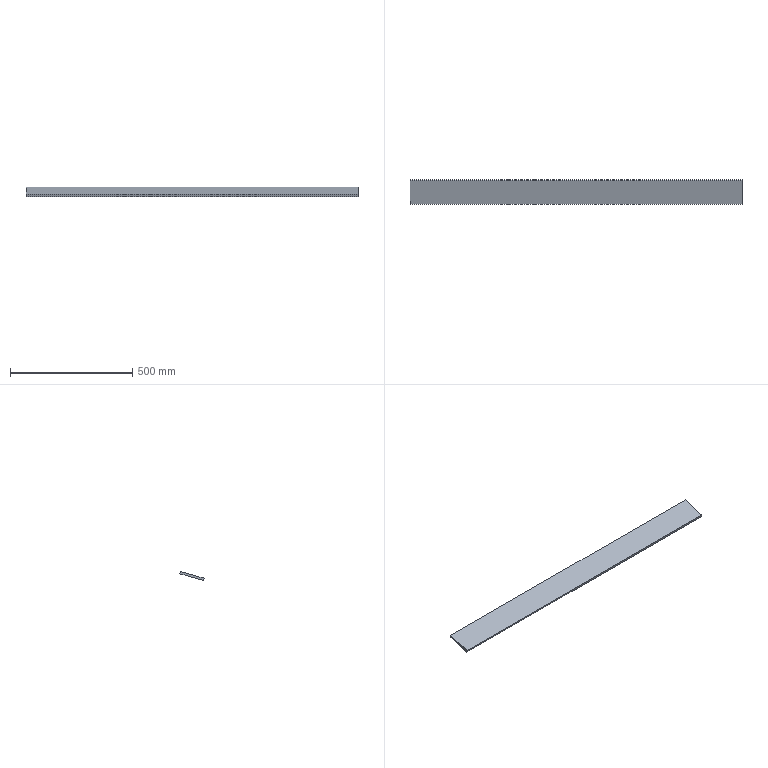Component | SolidWorks | Vezni lim 1-2 | 1 solid | 6 faces | box 1360 x 98.8 x 37.58 mm | volume 1360000 mm3 | plane 6
build123d program:
from build123d import *

# Parameters (mm, degrees)
SKETCH1_W           = 10
SKETCH1_H           = 100
BOSS_EXTRUDE1_DEPTH = 1360


with BuildPart() as part:
    # Sketch1 → Boss-Extrude1 (new body)
    with BuildSketch(Plane.XY):
        with Locations((-108.521, 110)):
            Rectangle(SKETCH1_W, SKETCH1_H)
    extrude(amount=-BOSS_EXTRUDE1_DEPTH)


solid = part.part

# Placed as in the assembly
solid = solid.moved(Location((-1313.6, 1002.358, 806.215), (16.245, -90, 0)))
STEP:
#1=CARTESIAN_POINT('',(1.827,42.981,28.111));
#2=VERTEX_POINT('',#1);
#3=CARTESIAN_POINT('',(1.827,46.761,29.212));
#4=VERTEX_POINT('',#3);
#5=CARTESIAN_POINT('',(1.827,46.761,29.212));
#6=DIRECTION('',(-0.,0.9601,0.2797));
#7=VECTOR('',#6,39.37);
#8=LINE('',#5,#7);
#9=EDGE_CURVE('',#2,#4,#8,.T.);
#10=ORIENTED_EDGE('',*,*,#9,.F.);
#11=CARTESIAN_POINT('',(-51.717,42.981,28.111));
#12=VERTEX_POINT('',#11);
#13=CARTESIAN_POINT('',(-51.717,42.981,28.111));
#14=DIRECTION('',(1.,0.,0.));
#15=VECTOR('',#14,39.37);
#16=LINE('',#13,#15);
#17=EDGE_CURVE('',#12,#2,#16,.T.);
#18=ORIENTED_EDGE('',*,*,#17,.F.);
#19=CARTESIAN_POINT('',(-51.717,46.761,29.212));
#20=VERTEX_POINT('',#19);
#21=CARTESIAN_POINT('',(-51.717,46.761,29.212));
#22=DIRECTION('',(-0.,0.9601,0.2797));
#23=VECTOR('',#22,39.37);
#24=LINE('',#21,#23);
#25=EDGE_CURVE('',#12,#20,#24,.T.);
#26=ORIENTED_EDGE('',*,*,#25,.T.);
#27=CARTESIAN_POINT('',(-51.717,46.761,29.212));
#28=DIRECTION('',(1.,0.,0.));
#29=VECTOR('',#28,39.37);
#30=LINE('',#27,#29);
#31=EDGE_CURVE('',#20,#4,#30,.T.);
#32=ORIENTED_EDGE('',*,*,#31,.T.);
#33=EDGE_LOOP('',(#10,#18,#26,#32));
#34=FACE_OUTER_BOUND('',#33,.T.);
#35=CARTESIAN_POINT('',(-51.717,46.761,29.212));
#36=DIRECTION('',(0.,0.2797,-0.9601));
#37=DIRECTION('',(-1.,-0.,-0.));
#38=AXIS2_PLACEMENT_3D('',#35,#36,#37);
#39=PLANE('',#38);
#40=ADVANCED_FACE('',(#34),#39,.T.);
#41=CARTESIAN_POINT('',(1.827,42.871,28.489));
#42=VERTEX_POINT('',#41);
#43=CARTESIAN_POINT('',(1.827,42.981,28.111));
#44=DIRECTION('',(0.,0.2797,-0.9601));
#45=VECTOR('',#44,39.37);
#46=LINE('',#43,#45);
#47=EDGE_CURVE('',#42,#2,#46,.T.);
#48=ORIENTED_EDGE('',*,*,#47,.F.);
#49=CARTESIAN_POINT('',(-51.717,42.871,28.489));
#50=VERTEX_POINT('',#49);
#51=CARTESIAN_POINT('',(-51.717,42.871,28.489));
#52=DIRECTION('',(1.,0.,0.));
#53=VECTOR('',#52,39.37);
#54=LINE('',#51,#53);
#55=EDGE_CURVE('',#50,#42,#54,.T.);
#56=ORIENTED_EDGE('',*,*,#55,.F.);
#57=CARTESIAN_POINT('',(-51.717,42.981,28.111));
#58=DIRECTION('',(0.,0.2797,-0.9601));
#59=VECTOR('',#58,39.37);
#60=LINE('',#57,#59);
#61=EDGE_CURVE('',#50,#12,#60,.T.);
#62=ORIENTED_EDGE('',*,*,#61,.T.);
#63=ORIENTED_EDGE('',*,*,#17,.T.);
#64=EDGE_LOOP('',(#48,#56,#62,#63));
#65=FACE_OUTER_BOUND('',#64,.T.);
#66=CARTESIAN_POINT('',(-51.717,42.981,28.111));
#67=DIRECTION('',(0.,-0.9601,-0.2797));
#68=DIRECTION('',(-1.,-0.,-0.));
#69=AXIS2_PLACEMENT_3D('',#66,#67,#68);
#70=PLANE('',#69);
#71=ADVANCED_FACE('',(#65),#70,.T.);
#72=CARTESIAN_POINT('',(1.827,46.651,29.59));
#73=VERTEX_POINT('',#72);
#74=CARTESIAN_POINT('',(1.827,46.651,29.59));
#75=DIRECTION('',(0.,-0.9601,-0.2797));
#76=VECTOR('',#75,39.37);
#77=LINE('',#74,#76);
#78=EDGE_CURVE('',#73,#42,#77,.T.);
#79=ORIENTED_EDGE('',*,*,#78,.F.);
#80=CARTESIAN_POINT('',(-51.717,46.651,29.59));
#81=VERTEX_POINT('',#80);
#82=CARTESIAN_POINT('',(-51.717,46.651,29.59));
#83=DIRECTION('',(1.,0.,0.));
#84=VECTOR('',#83,39.37);
#85=LINE('',#82,#84);
#86=EDGE_CURVE('',#81,#73,#85,.T.);
#87=ORIENTED_EDGE('',*,*,#86,.F.);
#88=CARTESIAN_POINT('',(-51.717,46.651,29.59));
#89=DIRECTION('',(0.,-0.9601,-0.2797));
#90=VECTOR('',#89,39.37);
#91=LINE('',#88,#90);
#92=EDGE_CURVE('',#81,#50,#91,.T.);
#93=ORIENTED_EDGE('',*,*,#92,.T.);
#94=ORIENTED_EDGE('',*,*,#55,.T.);
#95=EDGE_LOOP('',(#79,#87,#93,#94));
#96=FACE_OUTER_BOUND('',#95,.T.);
#97=CARTESIAN_POINT('',(-51.717,46.651,29.59));
#98=DIRECTION('',(-0.,-0.2797,0.9601));
#99=DIRECTION('',(0.,-0.9601,-0.2797));
#100=AXIS2_PLACEMENT_3D('',#97,#98,#99);
#101=PLANE('',#100);
#102=ADVANCED_FACE('',(#96),#101,.T.);
#103=CARTESIAN_POINT('',(1.827,46.761,29.212));
#104=DIRECTION('',(-0.,-0.2797,0.9601));
#105=VECTOR('',#104,39.37);
#106=LINE('',#103,#105);
#107=EDGE_CURVE('',#4,#73,#106,.T.);
#108=ORIENTED_EDGE('',*,*,#107,.F.);
#109=ORIENTED_EDGE('',*,*,#31,.F.);
#110=CARTESIAN_POINT('',(-51.717,46.761,29.212));
#111=DIRECTION('',(-0.,-0.2797,0.9601));
#112=VECTOR('',#111,39.37);
#113=LINE('',#110,#112);
#114=EDGE_CURVE('',#20,#81,#113,.T.);
#115=ORIENTED_EDGE('',*,*,#114,.T.);
#116=ORIENTED_EDGE('',*,*,#86,.T.);
#117=EDGE_LOOP('',(#108,#109,#115,#116));
#118=FACE_OUTER_BOUND('',#117,.T.);
#119=CARTESIAN_POINT('',(-51.717,46.761,29.212));
#120=DIRECTION('',(-0.,0.9601,0.2797));
#121=DIRECTION('',(1.,0.,0.));
#122=AXIS2_PLACEMENT_3D('',#119,#120,#121);
#123=PLANE('',#122);
#124=ADVANCED_FACE('',(#118),#123,.T.);
#125=ORIENTED_EDGE('',*,*,#25,.F.);
#126=ORIENTED_EDGE('',*,*,#61,.F.);
#127=ORIENTED_EDGE('',*,*,#92,.F.);
#128=ORIENTED_EDGE('',*,*,#114,.F.);
#129=EDGE_LOOP('',(#125,#126,#127,#128));
#130=FACE_OUTER_BOUND('',#129,.T.);
#131=CARTESIAN_POINT('',(-51.717,41.853,23.537));
#132=DIRECTION('',(-1.,-0.,-0.));
#133=DIRECTION('',(-0.,-0.2797,0.9601));
#134=AXIS2_PLACEMENT_3D('',#131,#132,#133);
#135=PLANE('',#134);
#136=ADVANCED_FACE('',(#130),#135,.T.);
#137=ORIENTED_EDGE('',*,*,#9,.T.);
#138=ORIENTED_EDGE('',*,*,#107,.T.);
#139=ORIENTED_EDGE('',*,*,#78,.T.);
#140=ORIENTED_EDGE('',*,*,#47,.T.);
#141=EDGE_LOOP('',(#137,#138,#139,#140));
#142=FACE_OUTER_BOUND('',#141,.T.);
#143=CARTESIAN_POINT('',(1.827,41.853,23.537));
#144=DIRECTION('',(-1.,-0.,-0.));
#145=DIRECTION('',(-0.,-0.2797,0.9601));
#146=AXIS2_PLACEMENT_3D('',#143,#144,#145);
#147=PLANE('',#146);
#148=ADVANCED_FACE('',(#142),#147,.F.);
#149=CLOSED_SHELL('',(#40,#71,#102,#124,#136,#148));
#150=MANIFOLD_SOLID_BREP('',#149);
#151=CARTESIAN_POINT('',(0.,0.,0.));
#152=DIRECTION('',(0.,0.,1.));
#153=DIRECTION('',(1.,0.,0.));
#154=AXIS2_PLACEMENT_3D('',#151,#152,#153);
#155=(LENGTH_UNIT()NAMED_UNIT(*)SI_UNIT($,.METRE.));
#156=LENGTH_MEASURE_WITH_UNIT(LENGTH_MEASURE(0.0254),#155);
#157=DIMENSIONAL_EXPONENTS(1.,0.,0.,0.,0.,0.,0.);
#158=(CONVERSION_BASED_UNIT('',#156)LENGTH_UNIT()NAMED_UNIT(#157));
#159=UNCERTAINTY_MEASURE_WITH_UNIT(LENGTH_MEASURE(0.00001),#158,'','');
#160=(NAMED_UNIT(*)PLANE_ANGLE_UNIT()SI_UNIT($,.RADIAN.));
#161=(NAMED_UNIT(*)SI_UNIT($,.STERADIAN.)SOLID_ANGLE_UNIT());
#162=(GEOMETRIC_REPRESENTATION_CONTEXT(3)GLOBAL_UNCERTAINTY_ASSIGNED_CONTEXT((#159))GLOBAL_UNIT_ASSIGNED_CONTEXT((#158,#160,#161))REPRESENTATION_CONTEXT('',''));
#163=ADVANCED_BREP_SHAPE_REPRESENTATION('',(#150,#154),#162);
#164=COLOUR_RGB('',0.7922,0.8196,0.9333);
#165=FILL_AREA_STYLE_COLOUR('',#164);
#166=FILL_AREA_STYLE('',(#165));
#167=SURFACE_STYLE_FILL_AREA(#166);
#168=SURFACE_SIDE_STYLE('',(#167));
#169=SURFACE_STYLE_USAGE(.BOTH.,#168);
#170=PRESENTATION_STYLE_ASSIGNMENT((#169));
#171=STYLED_ITEM('',(#170),#150);
#172=PRESENTATION_LAYER_ASSIGNMENT('','',(#171));
#173=(LENGTH_UNIT()NAMED_UNIT(*)SI_UNIT($,.METRE.));
#174=LENGTH_MEASURE_WITH_UNIT(LENGTH_MEASURE(0.0254),#173);
#175=DIMENSIONAL_EXPONENTS(1.,0.,0.,0.,0.,0.,0.);
#176=(CONVERSION_BASED_UNIT('',#174)LENGTH_UNIT()NAMED_UNIT(#175));
#177=UNCERTAINTY_MEASURE_WITH_UNIT(LENGTH_MEASURE(0.00001),#176,'','');
#178=(NAMED_UNIT(*)PLANE_ANGLE_UNIT()SI_UNIT($,.RADIAN.));
#179=(NAMED_UNIT(*)SI_UNIT($,.STERADIAN.)SOLID_ANGLE_UNIT());
#180=(GEOMETRIC_REPRESENTATION_CONTEXT(3)GLOBAL_UNCERTAINTY_ASSIGNED_CONTEXT((#177))GLOBAL_UNIT_ASSIGNED_CONTEXT((#176,#178,#179))REPRESENTATION_CONTEXT('',''));
#181=MECHANICAL_DESIGN_GEOMETRIC_PRESENTATION_REPRESENTATION('',(#171),#180);